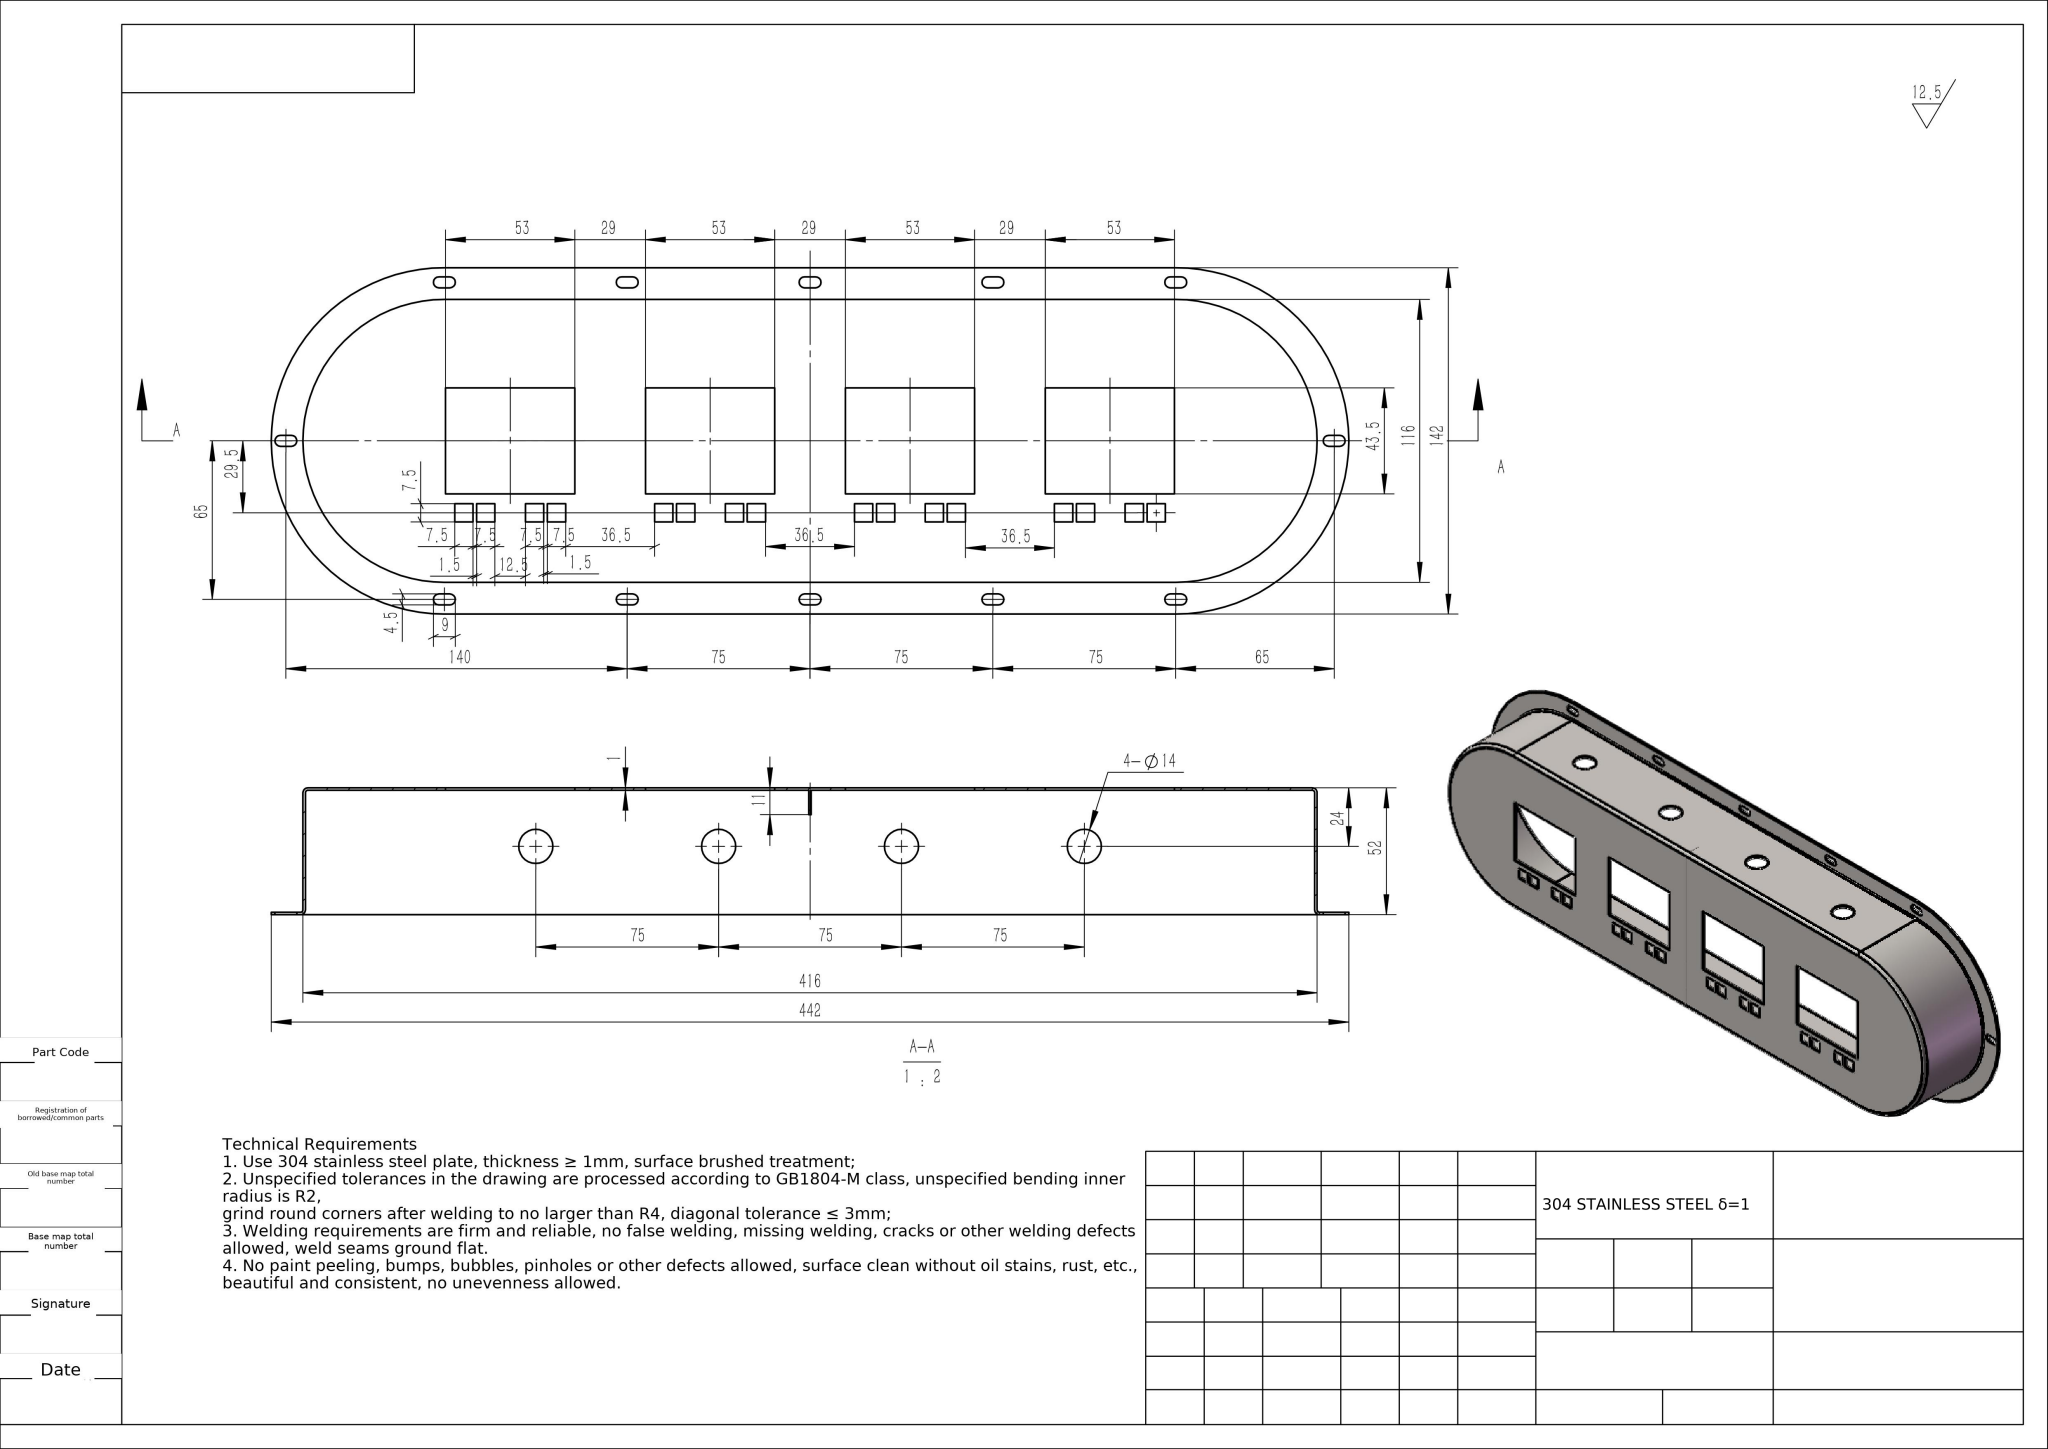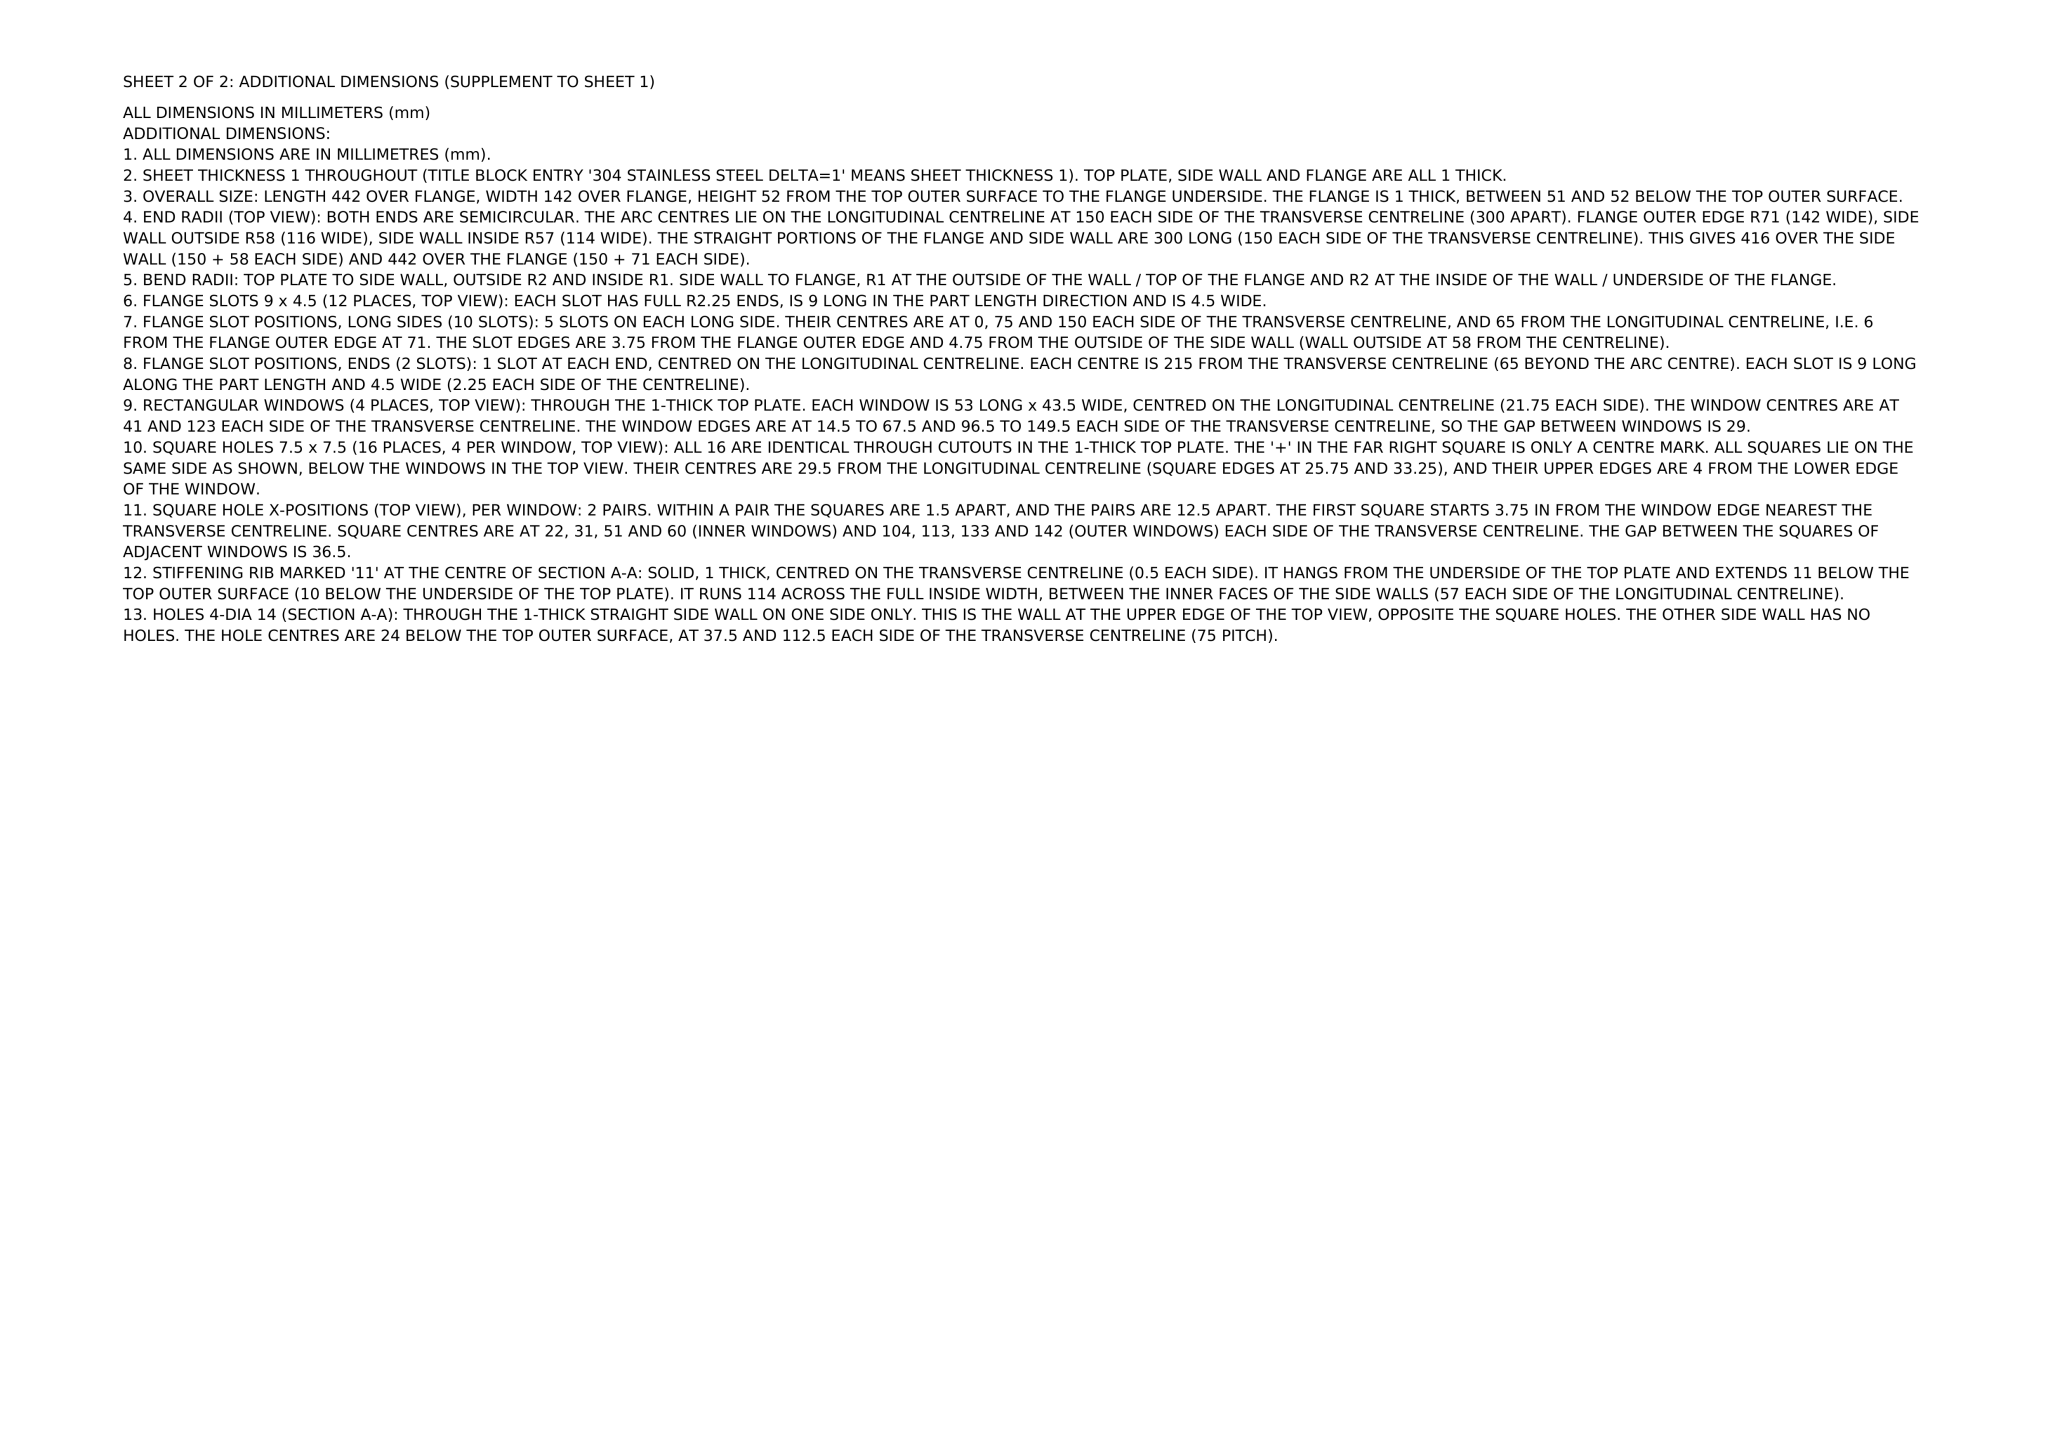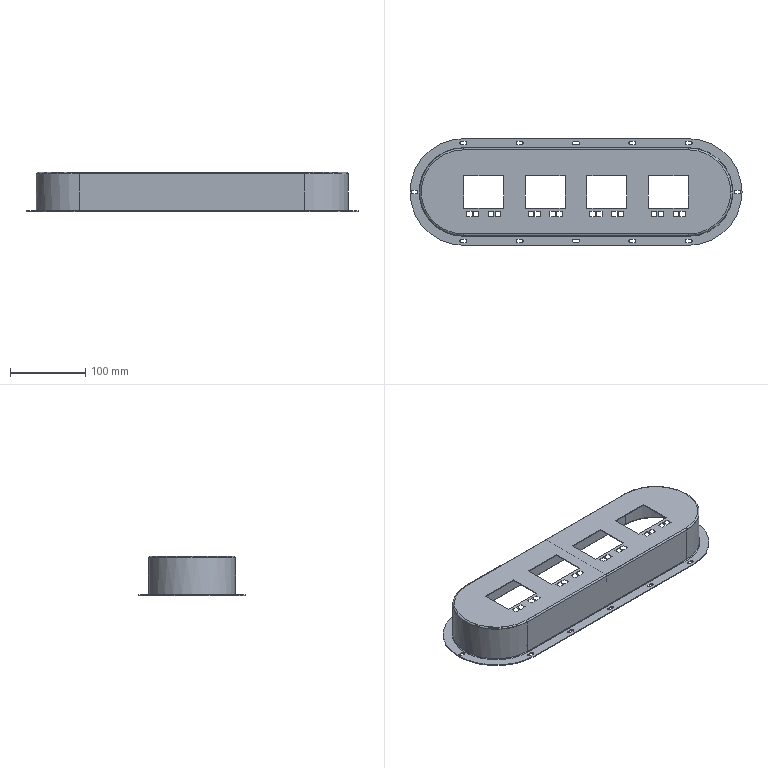Part | NX | mm | 1 solid | 193 faces | box 442 x 142 x 52 mm | volume 96192 mm3 | plane 118 | cylinder 63 | torus 12 | commonest cylinder face diameters 4.5 x36 14 x8 2 x6 4 x4 142 x3 114 x3 116 x3